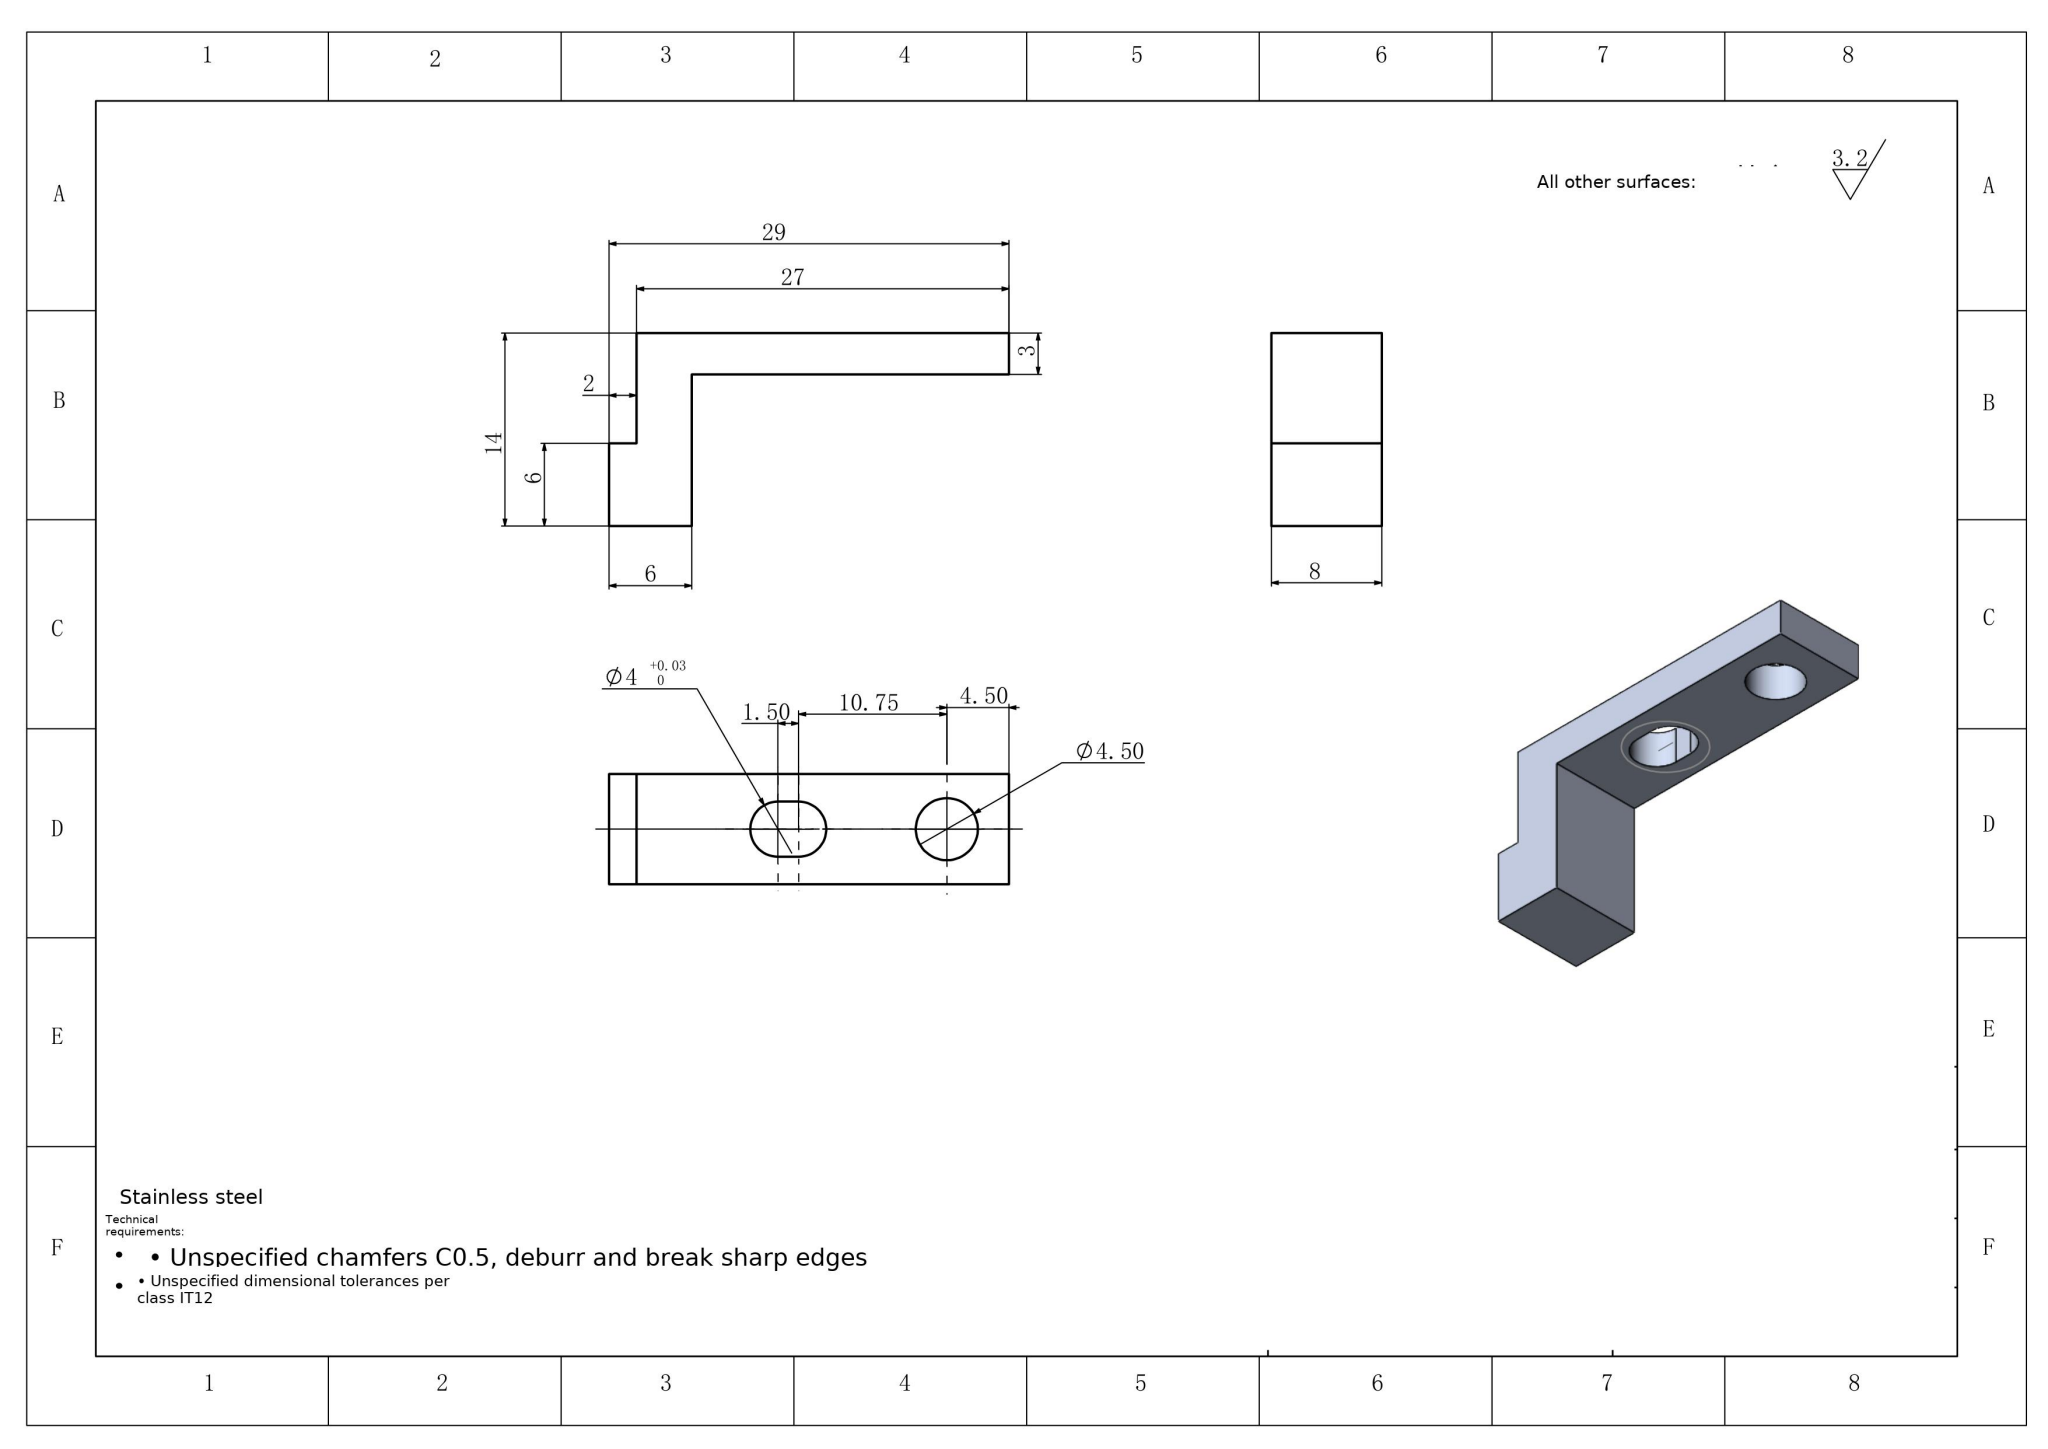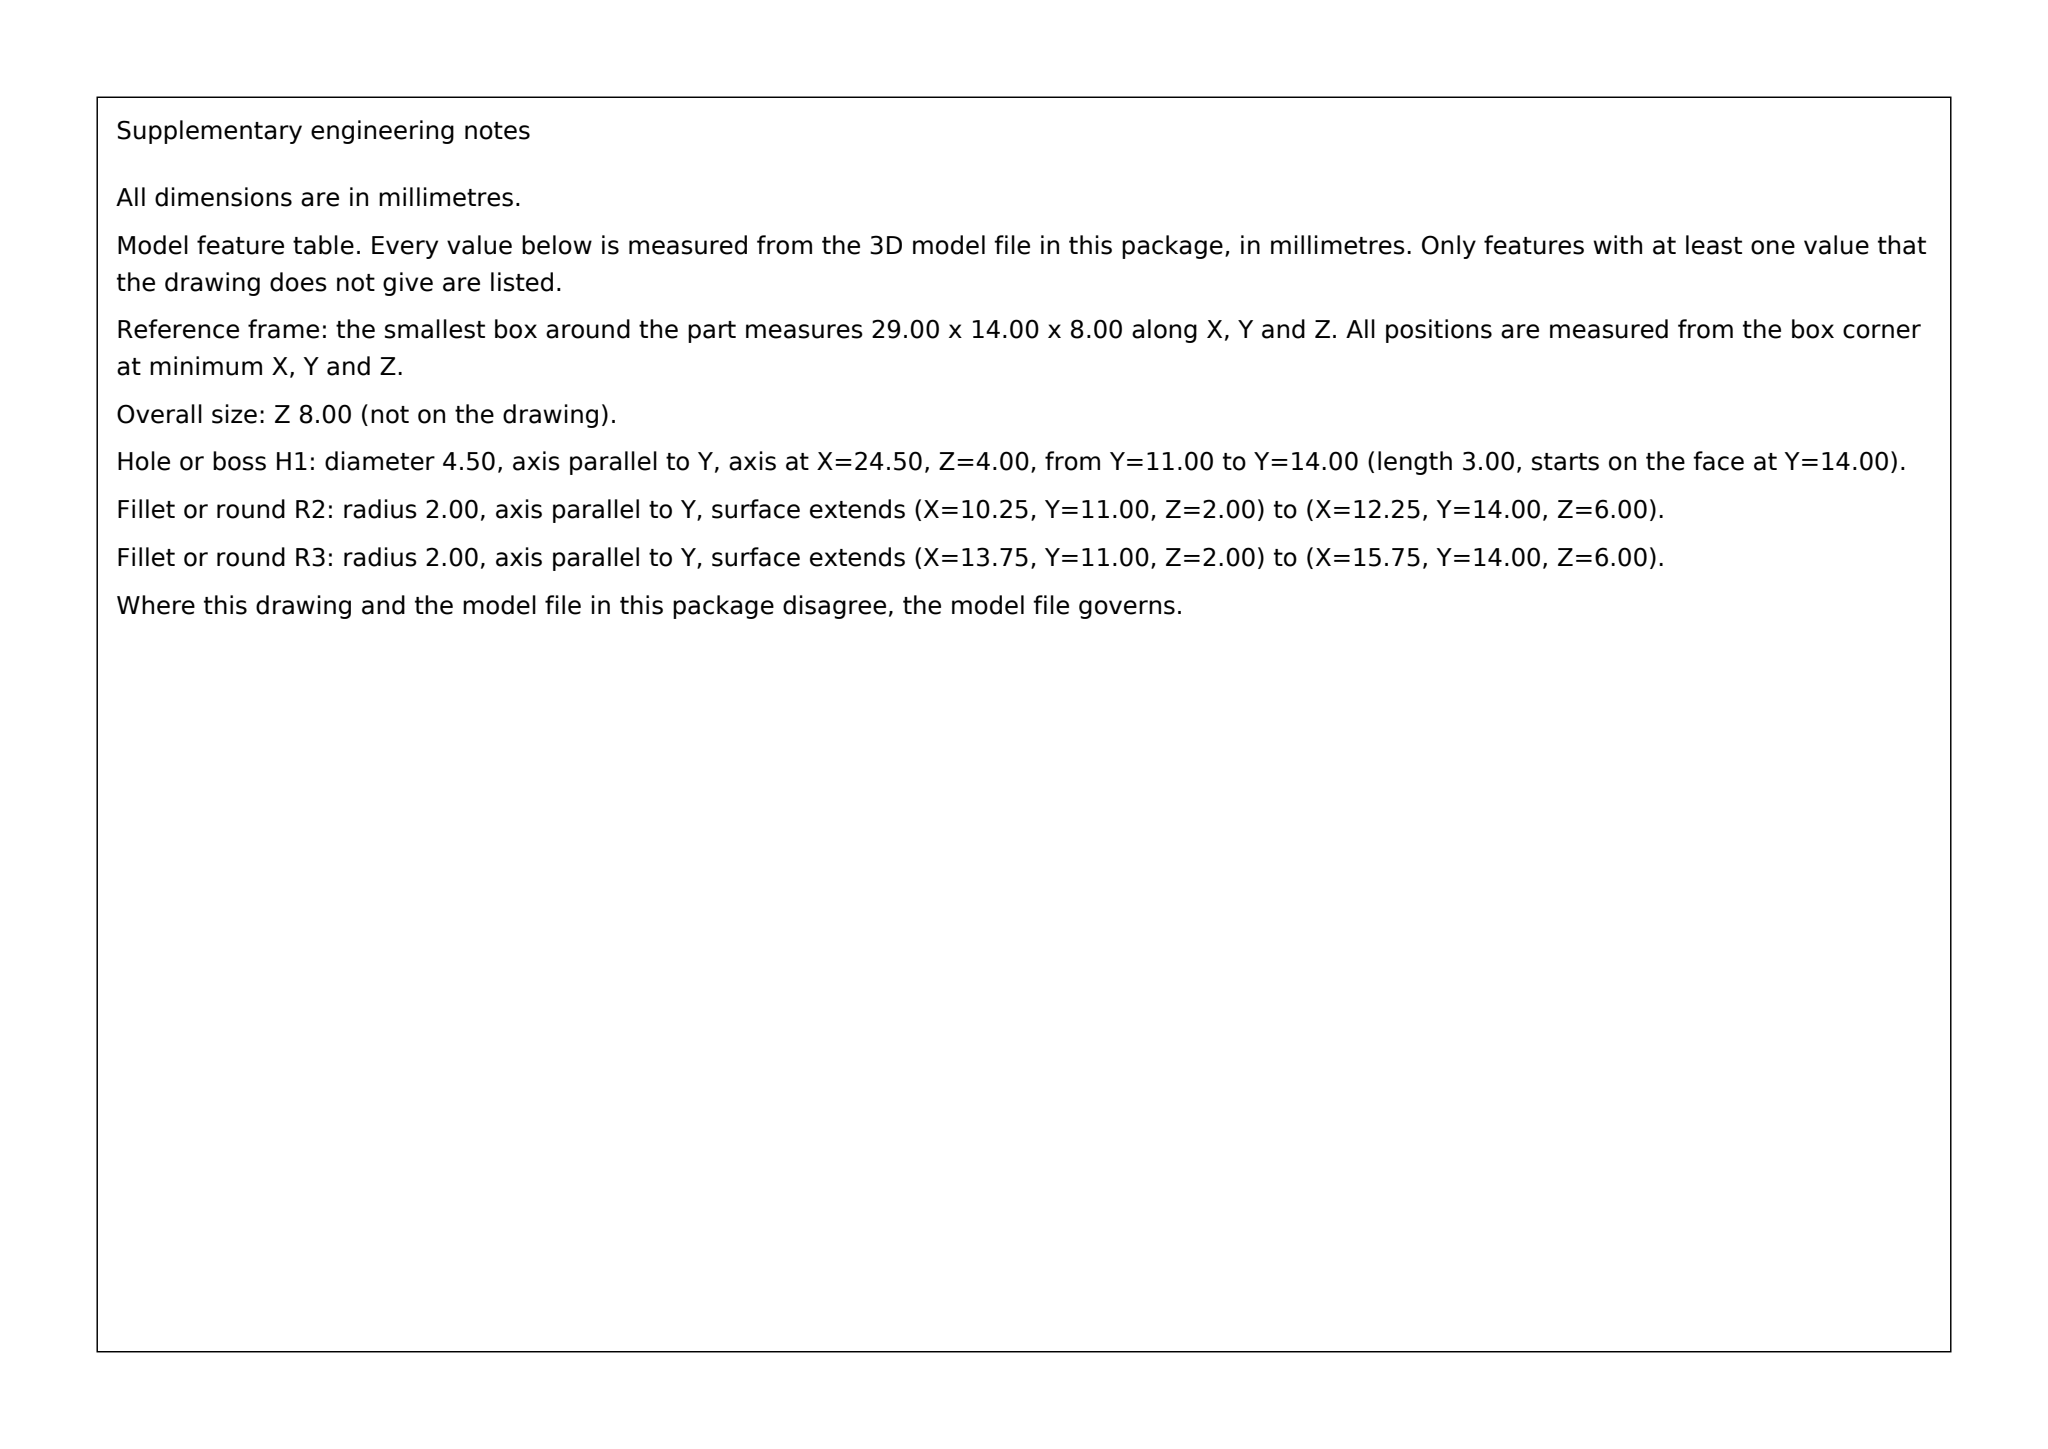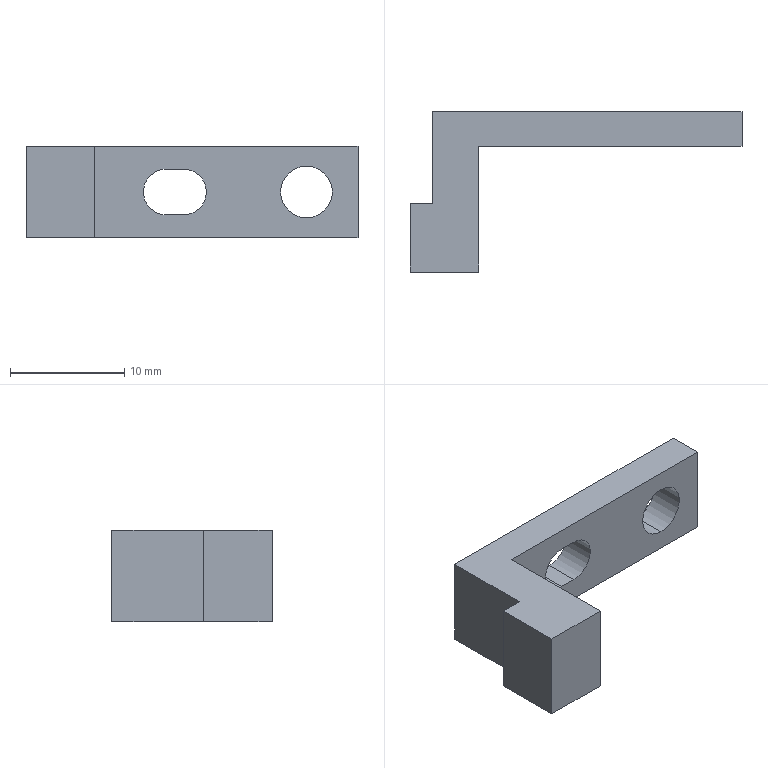Part | SolidWorks | mm | material Stainless steel | 1 solid | 16 faces | box 29 x 14 x 8 mm | volume 993 mm3 | plane 12 | cylinder 4 | commonest cylinder face diameters 4.5 x2 4 x2
build123d program:
from build123d import *

# Parameters (mm, degrees)
BOSS_EXTRUDE1_DEPTH = 4
SKETCH2_R           = 2.25
CUT_EXTRUDE1_DEPTH  = 30.428


with BuildPart() as part:
    # Sketch1 → Boss-Extrude1 (new, symmetric)
    with BuildSketch(Plane.XY):
        Polygon((0, 0), (0, -8), (-2, -8), (-2, -14), (4, -14), (4, -3), (27, -3), (27, 0), align=None)
    extrude(amount=BOSS_EXTRUDE1_DEPTH, both=True)

    # Sketch2 → Cut-Extrude1 (cut, through all)
    with BuildSketch(Plane.XZ.offset(3)):
        with Locations(Location((22.5, 0, 0), (0, 0, 270))):
            Circle(SKETCH2_R)
        with BuildLine():
            Line((10.25, 2), (11.75, 2))
            ThreePointArc((11.75, 2), (13.75, 0), (11.75, -2))
            Line((11.75, -2), (10.25, -2))
            ThreePointArc((10.25, -2), (8.25, 0), (10.25, 2))
        make_face()
    extrude(amount=-CUT_EXTRUDE1_DEPTH, mode=Mode.SUBTRACT)


solid = part.part
STEP:
#1=CARTESIAN_POINT('',(22.5,0.,2.25));
#2=VERTEX_POINT('',#1);
#3=CARTESIAN_POINT('',(22.5,0.,-2.25));
#4=VERTEX_POINT('',#3);
#5=CARTESIAN_POINT('',(22.5,0.,-0.));
#6=DIRECTION('',(0.,-1.,0.));
#7=DIRECTION('',(0.,0.,-1.));
#8=AXIS2_PLACEMENT_3D('',#5,#6,#7);
#9=CIRCLE('',#8,2.25);
#10=EDGE_CURVE('',#2,#4,#9,.T.);
#11=ORIENTED_EDGE('',*,*,#10,.F.);
#12=CARTESIAN_POINT('',(22.5,-3.,2.25));
#13=VERTEX_POINT('',#12);
#14=CARTESIAN_POINT('',(22.5,0.,2.25));
#15=DIRECTION('',(0.,-1.,0.));
#16=VECTOR('',#15,1000.);
#17=LINE('',#14,#16);
#18=EDGE_CURVE('',#2,#13,#17,.T.);
#19=ORIENTED_EDGE('',*,*,#18,.T.);
#20=CARTESIAN_POINT('',(22.5,-3.,-2.25));
#21=VERTEX_POINT('',#20);
#22=CARTESIAN_POINT('',(22.5,-3.,-0.));
#23=DIRECTION('',(0.,-1.,0.));
#24=DIRECTION('',(0.,0.,-1.));
#25=AXIS2_PLACEMENT_3D('',#22,#23,#24);
#26=CIRCLE('',#25,2.25);
#27=EDGE_CURVE('',#13,#21,#26,.T.);
#28=ORIENTED_EDGE('',*,*,#27,.T.);
#29=CARTESIAN_POINT('',(22.5,0.,-2.25));
#30=DIRECTION('',(0.,-1.,0.));
#31=VECTOR('',#30,1000.);
#32=LINE('',#29,#31);
#33=EDGE_CURVE('',#4,#21,#32,.T.);
#34=ORIENTED_EDGE('',*,*,#33,.F.);
#35=EDGE_LOOP('',(#11,#19,#28,#34));
#36=FACE_OUTER_BOUND('',#35,.T.);
#37=CARTESIAN_POINT('',(22.5,0.,-0.));
#38=DIRECTION('',(0.,-1.,0.));
#39=DIRECTION('',(0.,0.,-1.));
#40=AXIS2_PLACEMENT_3D('',#37,#38,#39);
#41=CYLINDRICAL_SURFACE('',#40,2.25);
#42=ADVANCED_FACE('',(#36),#41,.F.);
#43=CARTESIAN_POINT('',(11.75,0.,2.));
#44=VERTEX_POINT('',#43);
#45=CARTESIAN_POINT('',(10.25,0.,2.));
#46=VERTEX_POINT('',#45);
#47=CARTESIAN_POINT('',(10.25,0.,2.));
#48=DIRECTION('',(-1.,0.,-0.));
#49=VECTOR('',#48,1000.);
#50=LINE('',#47,#49);
#51=EDGE_CURVE('',#44,#46,#50,.T.);
#52=ORIENTED_EDGE('',*,*,#51,.T.);
#53=CARTESIAN_POINT('',(10.25,0.,-2.));
#54=VERTEX_POINT('',#53);
#55=CARTESIAN_POINT('',(10.25,0.,-0.));
#56=DIRECTION('',(0.,-1.,0.));
#57=DIRECTION('',(0.,0.,-1.));
#58=AXIS2_PLACEMENT_3D('',#55,#56,#57);
#59=CIRCLE('',#58,2.);
#60=EDGE_CURVE('',#46,#54,#59,.T.);
#61=ORIENTED_EDGE('',*,*,#60,.T.);
#62=CARTESIAN_POINT('',(11.75,0.,-2.));
#63=VERTEX_POINT('',#62);
#64=CARTESIAN_POINT('',(10.25,0.,-2.));
#65=DIRECTION('',(1.,0.,0.));
#66=VECTOR('',#65,1000.);
#67=LINE('',#64,#66);
#68=EDGE_CURVE('',#54,#63,#67,.T.);
#69=ORIENTED_EDGE('',*,*,#68,.T.);
#70=CARTESIAN_POINT('',(11.75,0.,-0.));
#71=DIRECTION('',(0.,-1.,0.));
#72=DIRECTION('',(0.,0.,-1.));
#73=AXIS2_PLACEMENT_3D('',#70,#71,#72);
#74=CIRCLE('',#73,2.);
#75=EDGE_CURVE('',#63,#44,#74,.T.);
#76=ORIENTED_EDGE('',*,*,#75,.T.);
#77=EDGE_LOOP('',(#52,#61,#69,#76));
#78=FACE_BOUND('',#77,.T.);
#79=CARTESIAN_POINT('',(22.5,0.,-0.));
#80=DIRECTION('',(0.,-1.,0.));
#81=DIRECTION('',(0.,0.,-1.));
#82=AXIS2_PLACEMENT_3D('',#79,#80,#81);
#83=CIRCLE('',#82,2.25);
#84=EDGE_CURVE('',#4,#2,#83,.T.);
#85=ORIENTED_EDGE('',*,*,#84,.T.);
#86=ORIENTED_EDGE('',*,*,#10,.T.);
#87=EDGE_LOOP('',(#85,#86));
#88=FACE_BOUND('',#87,.T.);
#89=CARTESIAN_POINT('',(27.,0.,-4.));
#90=VERTEX_POINT('',#89);
#91=CARTESIAN_POINT('',(0.,0.,-4.));
#92=VERTEX_POINT('',#91);
#93=CARTESIAN_POINT('',(27.,0.,-4.));
#94=DIRECTION('',(-1.,-0.,0.));
#95=VECTOR('',#94,1000.);
#96=LINE('',#93,#95);
#97=EDGE_CURVE('',#90,#92,#96,.T.);
#98=ORIENTED_EDGE('',*,*,#97,.T.);
#99=CARTESIAN_POINT('',(0.,0.,4.));
#100=VERTEX_POINT('',#99);
#101=CARTESIAN_POINT('',(0.,0.,4.));
#102=DIRECTION('',(0.,0.,-1.));
#103=VECTOR('',#102,1000.);
#104=LINE('',#101,#103);
#105=EDGE_CURVE('',#100,#92,#104,.T.);
#106=ORIENTED_EDGE('',*,*,#105,.F.);
#107=CARTESIAN_POINT('',(27.,0.,4.));
#108=VERTEX_POINT('',#107);
#109=CARTESIAN_POINT('',(27.,0.,4.));
#110=DIRECTION('',(-1.,-0.,0.));
#111=VECTOR('',#110,1000.);
#112=LINE('',#109,#111);
#113=EDGE_CURVE('',#108,#100,#112,.T.);
#114=ORIENTED_EDGE('',*,*,#113,.F.);
#115=CARTESIAN_POINT('',(27.,0.,4.));
#116=DIRECTION('',(0.,0.,-1.));
#117=VECTOR('',#116,1000.);
#118=LINE('',#115,#117);
#119=EDGE_CURVE('',#108,#90,#118,.T.);
#120=ORIENTED_EDGE('',*,*,#119,.T.);
#121=EDGE_LOOP('',(#98,#106,#114,#120));
#122=FACE_OUTER_BOUND('',#121,.T.);
#123=CARTESIAN_POINT('',(27.,0.,4.));
#124=DIRECTION('',(0.,-1.,0.));
#125=DIRECTION('',(1.,0.,0.));
#126=AXIS2_PLACEMENT_3D('',#123,#124,#125);
#127=PLANE('',#126);
#128=ADVANCED_FACE('',(#78,#88,#122),#127,.F.);
#129=CARTESIAN_POINT('',(0.,-8.,-4.));
#130=VERTEX_POINT('',#129);
#131=CARTESIAN_POINT('',(0.,0.,-4.));
#132=DIRECTION('',(0.,-1.,0.));
#133=VECTOR('',#132,1000.);
#134=LINE('',#131,#133);
#135=EDGE_CURVE('',#92,#130,#134,.T.);
#136=ORIENTED_EDGE('',*,*,#135,.T.);
#137=CARTESIAN_POINT('',(0.,-8.,4.));
#138=VERTEX_POINT('',#137);
#139=CARTESIAN_POINT('',(0.,-8.,4.));
#140=DIRECTION('',(0.,0.,-1.));
#141=VECTOR('',#140,1000.);
#142=LINE('',#139,#141);
#143=EDGE_CURVE('',#138,#130,#142,.T.);
#144=ORIENTED_EDGE('',*,*,#143,.F.);
#145=CARTESIAN_POINT('',(0.,0.,4.));
#146=DIRECTION('',(0.,-1.,0.));
#147=VECTOR('',#146,1000.);
#148=LINE('',#145,#147);
#149=EDGE_CURVE('',#100,#138,#148,.T.);
#150=ORIENTED_EDGE('',*,*,#149,.F.);
#151=ORIENTED_EDGE('',*,*,#105,.T.);
#152=EDGE_LOOP('',(#136,#144,#150,#151));
#153=FACE_OUTER_BOUND('',#152,.T.);
#154=CARTESIAN_POINT('',(0.,0.,4.));
#155=DIRECTION('',(1.,0.,0.));
#156=DIRECTION('',(-0.,1.,0.));
#157=AXIS2_PLACEMENT_3D('',#154,#155,#156);
#158=PLANE('',#157);
#159=ADVANCED_FACE('',(#153),#158,.F.);
#160=CARTESIAN_POINT('',(-2.,-8.,-4.));
#161=VERTEX_POINT('',#160);
#162=CARTESIAN_POINT('',(0.,-8.,-4.));
#163=DIRECTION('',(-1.,0.,0.));
#164=VECTOR('',#163,1000.);
#165=LINE('',#162,#164);
#166=EDGE_CURVE('',#130,#161,#165,.T.);
#167=ORIENTED_EDGE('',*,*,#166,.T.);
#168=CARTESIAN_POINT('',(-2.,-8.,4.));
#169=VERTEX_POINT('',#168);
#170=CARTESIAN_POINT('',(-2.,-8.,4.));
#171=DIRECTION('',(0.,0.,-1.));
#172=VECTOR('',#171,1000.);
#173=LINE('',#170,#172);
#174=EDGE_CURVE('',#169,#161,#173,.T.);
#175=ORIENTED_EDGE('',*,*,#174,.F.);
#176=CARTESIAN_POINT('',(0.,-8.,4.));
#177=DIRECTION('',(-1.,0.,0.));
#178=VECTOR('',#177,1000.);
#179=LINE('',#176,#178);
#180=EDGE_CURVE('',#138,#169,#179,.T.);
#181=ORIENTED_EDGE('',*,*,#180,.F.);
#182=ORIENTED_EDGE('',*,*,#143,.T.);
#183=EDGE_LOOP('',(#167,#175,#181,#182));
#184=FACE_OUTER_BOUND('',#183,.T.);
#185=CARTESIAN_POINT('',(0.,-8.,4.));
#186=DIRECTION('',(0.,-1.,0.));
#187=DIRECTION('',(0.,0.,-1.));
#188=AXIS2_PLACEMENT_3D('',#185,#186,#187);
#189=PLANE('',#188);
#190=ADVANCED_FACE('',(#184),#189,.F.);
#191=CARTESIAN_POINT('',(-2.,-14.,-4.));
#192=VERTEX_POINT('',#191);
#193=CARTESIAN_POINT('',(-2.,-8.,-4.));
#194=DIRECTION('',(0.,-1.,0.));
#195=VECTOR('',#194,1000.);
#196=LINE('',#193,#195);
#197=EDGE_CURVE('',#161,#192,#196,.T.);
#198=ORIENTED_EDGE('',*,*,#197,.T.);
#199=CARTESIAN_POINT('',(-2.,-14.,4.));
#200=VERTEX_POINT('',#199);
#201=CARTESIAN_POINT('',(-2.,-14.,4.));
#202=DIRECTION('',(0.,0.,-1.));
#203=VECTOR('',#202,1000.);
#204=LINE('',#201,#203);
#205=EDGE_CURVE('',#200,#192,#204,.T.);
#206=ORIENTED_EDGE('',*,*,#205,.F.);
#207=CARTESIAN_POINT('',(-2.,-8.,4.));
#208=DIRECTION('',(0.,-1.,0.));
#209=VECTOR('',#208,1000.);
#210=LINE('',#207,#209);
#211=EDGE_CURVE('',#169,#200,#210,.T.);
#212=ORIENTED_EDGE('',*,*,#211,.F.);
#213=ORIENTED_EDGE('',*,*,#174,.T.);
#214=EDGE_LOOP('',(#198,#206,#212,#213));
#215=FACE_OUTER_BOUND('',#214,.T.);
#216=CARTESIAN_POINT('',(-2.,-8.,4.));
#217=DIRECTION('',(1.,0.,0.));
#218=DIRECTION('',(-0.,1.,0.));
#219=AXIS2_PLACEMENT_3D('',#216,#217,#218);
#220=PLANE('',#219);
#221=ADVANCED_FACE('',(#215),#220,.F.);
#222=CARTESIAN_POINT('',(4.,-14.,-4.));
#223=VERTEX_POINT('',#222);
#224=CARTESIAN_POINT('',(-2.,-14.,-4.));
#225=DIRECTION('',(1.,0.,0.));
#226=VECTOR('',#225,1000.);
#227=LINE('',#224,#226);
#228=EDGE_CURVE('',#192,#223,#227,.T.);
#229=ORIENTED_EDGE('',*,*,#228,.T.);
#230=CARTESIAN_POINT('',(4.,-14.,4.));
#231=VERTEX_POINT('',#230);
#232=CARTESIAN_POINT('',(4.,-14.,4.));
#233=DIRECTION('',(0.,0.,-1.));
#234=VECTOR('',#233,1000.);
#235=LINE('',#232,#234);
#236=EDGE_CURVE('',#231,#223,#235,.T.);
#237=ORIENTED_EDGE('',*,*,#236,.F.);
#238=CARTESIAN_POINT('',(-2.,-14.,4.));
#239=DIRECTION('',(1.,0.,0.));
#240=VECTOR('',#239,1000.);
#241=LINE('',#238,#240);
#242=EDGE_CURVE('',#200,#231,#241,.T.);
#243=ORIENTED_EDGE('',*,*,#242,.F.);
#244=ORIENTED_EDGE('',*,*,#205,.T.);
#245=EDGE_LOOP('',(#229,#237,#243,#244));
#246=FACE_OUTER_BOUND('',#245,.T.);
#247=CARTESIAN_POINT('',(-2.,-14.,4.));
#248=DIRECTION('',(0.,1.,0.));
#249=DIRECTION('',(0.,0.,1.));
#250=AXIS2_PLACEMENT_3D('',#247,#248,#249);
#251=PLANE('',#250);
#252=ADVANCED_FACE('',(#246),#251,.F.);
#253=CARTESIAN_POINT('',(4.,-3.,-4.));
#254=VERTEX_POINT('',#253);
#255=CARTESIAN_POINT('',(4.,-14.,-4.));
#256=DIRECTION('',(0.,1.,0.));
#257=VECTOR('',#256,1000.);
#258=LINE('',#255,#257);
#259=EDGE_CURVE('',#223,#254,#258,.T.);
#260=ORIENTED_EDGE('',*,*,#259,.T.);
#261=CARTESIAN_POINT('',(4.,-3.,4.));
#262=VERTEX_POINT('',#261);
#263=CARTESIAN_POINT('',(4.,-3.,4.));
#264=DIRECTION('',(0.,0.,-1.));
#265=VECTOR('',#264,1000.);
#266=LINE('',#263,#265);
#267=EDGE_CURVE('',#262,#254,#266,.T.);
#268=ORIENTED_EDGE('',*,*,#267,.F.);
#269=CARTESIAN_POINT('',(4.,-14.,4.));
#270=DIRECTION('',(0.,1.,0.));
#271=VECTOR('',#270,1000.);
#272=LINE('',#269,#271);
#273=EDGE_CURVE('',#231,#262,#272,.T.);
#274=ORIENTED_EDGE('',*,*,#273,.F.);
#275=ORIENTED_EDGE('',*,*,#236,.T.);
#276=EDGE_LOOP('',(#260,#268,#274,#275));
#277=FACE_OUTER_BOUND('',#276,.T.);
#278=CARTESIAN_POINT('',(4.,-14.,4.));
#279=DIRECTION('',(-1.,0.,0.));
#280=DIRECTION('',(0.,0.,1.));
#281=AXIS2_PLACEMENT_3D('',#278,#279,#280);
#282=PLANE('',#281);
#283=ADVANCED_FACE('',(#277),#282,.F.);
#284=CARTESIAN_POINT('',(10.25,-3.,-2.));
#285=VERTEX_POINT('',#284);
#286=CARTESIAN_POINT('',(11.75,-3.,-2.));
#287=VERTEX_POINT('',#286);
#288=CARTESIAN_POINT('',(10.25,-3.,-2.));
#289=DIRECTION('',(1.,0.,0.));
#290=VECTOR('',#289,1000.);
#291=LINE('',#288,#290);
#292=EDGE_CURVE('',#285,#287,#291,.T.);
#293=ORIENTED_EDGE('',*,*,#292,.F.);
#294=CARTESIAN_POINT('',(10.25,-3.,2.));
#295=VERTEX_POINT('',#294);
#296=CARTESIAN_POINT('',(10.25,-3.,-0.));
#297=DIRECTION('',(0.,-1.,0.));
#298=DIRECTION('',(0.,0.,-1.));
#299=AXIS2_PLACEMENT_3D('',#296,#297,#298);
#300=CIRCLE('',#299,2.);
#301=EDGE_CURVE('',#295,#285,#300,.T.);
#302=ORIENTED_EDGE('',*,*,#301,.F.);
#303=CARTESIAN_POINT('',(11.75,-3.,2.));
#304=VERTEX_POINT('',#303);
#305=CARTESIAN_POINT('',(10.25,-3.,2.));
#306=DIRECTION('',(-1.,0.,-0.));
#307=VECTOR('',#306,1000.);
#308=LINE('',#305,#307);
#309=EDGE_CURVE('',#304,#295,#308,.T.);
#310=ORIENTED_EDGE('',*,*,#309,.F.);
#311=CARTESIAN_POINT('',(11.75,-3.,-0.));
#312=DIRECTION('',(0.,-1.,0.));
#313=DIRECTION('',(0.,0.,-1.));
#314=AXIS2_PLACEMENT_3D('',#311,#312,#313);
#315=CIRCLE('',#314,2.);
#316=EDGE_CURVE('',#287,#304,#315,.T.);
#317=ORIENTED_EDGE('',*,*,#316,.F.);
#318=EDGE_LOOP('',(#293,#302,#310,#317));
#319=FACE_BOUND('',#318,.T.);
#320=CARTESIAN_POINT('',(22.5,-3.,-0.));
#321=DIRECTION('',(0.,-1.,0.));
#322=DIRECTION('',(0.,0.,-1.));
#323=AXIS2_PLACEMENT_3D('',#320,#321,#322);
#324=CIRCLE('',#323,2.25);
#325=EDGE_CURVE('',#21,#13,#324,.T.);
#326=ORIENTED_EDGE('',*,*,#325,.F.);
#327=ORIENTED_EDGE('',*,*,#27,.F.);
#328=EDGE_LOOP('',(#326,#327));
#329=FACE_BOUND('',#328,.T.);
#330=CARTESIAN_POINT('',(27.,-3.,-4.));
#331=VERTEX_POINT('',#330);
#332=CARTESIAN_POINT('',(4.,-3.,-4.));
#333=DIRECTION('',(1.,0.,0.));
#334=VECTOR('',#333,1000.);
#335=LINE('',#332,#334);
#336=EDGE_CURVE('',#254,#331,#335,.T.);
#337=ORIENTED_EDGE('',*,*,#336,.T.);
#338=CARTESIAN_POINT('',(27.,-3.,4.));
#339=VERTEX_POINT('',#338);
#340=CARTESIAN_POINT('',(27.,-3.,4.));
#341=DIRECTION('',(0.,0.,-1.));
#342=VECTOR('',#341,1000.);
#343=LINE('',#340,#342);
#344=EDGE_CURVE('',#339,#331,#343,.T.);
#345=ORIENTED_EDGE('',*,*,#344,.F.);
#346=CARTESIAN_POINT('',(4.,-3.,4.));
#347=DIRECTION('',(1.,0.,0.));
#348=VECTOR('',#347,1000.);
#349=LINE('',#346,#348);
#350=EDGE_CURVE('',#262,#339,#349,.T.);
#351=ORIENTED_EDGE('',*,*,#350,.F.);
#352=ORIENTED_EDGE('',*,*,#267,.T.);
#353=EDGE_LOOP('',(#337,#345,#351,#352));
#354=FACE_OUTER_BOUND('',#353,.T.);
#355=CARTESIAN_POINT('',(4.,-3.,4.));
#356=DIRECTION('',(-0.,1.,0.));
#357=DIRECTION('',(-1.,-0.,0.));
#358=AXIS2_PLACEMENT_3D('',#355,#356,#357);
#359=PLANE('',#358);
#360=ADVANCED_FACE('',(#319,#329,#354),#359,.F.);
#361=CARTESIAN_POINT('',(27.,-3.,-4.));
#362=DIRECTION('',(0.,1.,0.));
#363=VECTOR('',#362,1000.);
#364=LINE('',#361,#363);
#365=EDGE_CURVE('',#331,#90,#364,.T.);
#366=ORIENTED_EDGE('',*,*,#365,.T.);
#367=ORIENTED_EDGE('',*,*,#119,.F.);
#368=CARTESIAN_POINT('',(27.,-3.,4.));
#369=DIRECTION('',(0.,1.,0.));
#370=VECTOR('',#369,1000.);
#371=LINE('',#368,#370);
#372=EDGE_CURVE('',#339,#108,#371,.T.);
#373=ORIENTED_EDGE('',*,*,#372,.F.);
#374=ORIENTED_EDGE('',*,*,#344,.T.);
#375=EDGE_LOOP('',(#366,#367,#373,#374));
#376=FACE_OUTER_BOUND('',#375,.T.);
#377=CARTESIAN_POINT('',(27.,-3.,4.));
#378=DIRECTION('',(-1.,0.,0.));
#379=DIRECTION('',(0.,0.,1.));
#380=AXIS2_PLACEMENT_3D('',#377,#378,#379);
#381=PLANE('',#380);
#382=ADVANCED_FACE('',(#376),#381,.F.);
#383=ORIENTED_EDGE('',*,*,#113,.T.);
#384=ORIENTED_EDGE('',*,*,#149,.T.);
#385=ORIENTED_EDGE('',*,*,#180,.T.);
#386=ORIENTED_EDGE('',*,*,#211,.T.);
#387=ORIENTED_EDGE('',*,*,#242,.T.);
#388=ORIENTED_EDGE('',*,*,#273,.T.);
#389=ORIENTED_EDGE('',*,*,#350,.T.);
#390=ORIENTED_EDGE('',*,*,#372,.T.);
#391=EDGE_LOOP('',(#383,#384,#385,#386,#387,#388,#389,#390));
#392=FACE_OUTER_BOUND('',#391,.T.);
#393=CARTESIAN_POINT('',(0.,0.,4.));
#394=DIRECTION('',(0.,0.,1.));
#395=DIRECTION('',(1.,0.,0.));
#396=AXIS2_PLACEMENT_3D('',#393,#394,#395);
#397=PLANE('',#396);
#398=ADVANCED_FACE('',(#392),#397,.T.);
#399=ORIENTED_EDGE('',*,*,#97,.F.);
#400=ORIENTED_EDGE('',*,*,#365,.F.);
#401=ORIENTED_EDGE('',*,*,#336,.F.);
#402=ORIENTED_EDGE('',*,*,#259,.F.);
#403=ORIENTED_EDGE('',*,*,#228,.F.);
#404=ORIENTED_EDGE('',*,*,#197,.F.);
#405=ORIENTED_EDGE('',*,*,#166,.F.);
#406=ORIENTED_EDGE('',*,*,#135,.F.);
#407=EDGE_LOOP('',(#399,#400,#401,#402,#403,#404,#405,#406));
#408=FACE_OUTER_BOUND('',#407,.T.);
#409=CARTESIAN_POINT('',(0.,0.,-4.));
#410=DIRECTION('',(0.,0.,1.));
#411=DIRECTION('',(1.,0.,0.));
#412=AXIS2_PLACEMENT_3D('',#409,#410,#411);
#413=PLANE('',#412);
#414=ADVANCED_FACE('',(#408),#413,.F.);
#415=ORIENTED_EDGE('',*,*,#18,.F.);
#416=ORIENTED_EDGE('',*,*,#84,.F.);
#417=ORIENTED_EDGE('',*,*,#33,.T.);
#418=ORIENTED_EDGE('',*,*,#325,.T.);
#419=EDGE_LOOP('',(#415,#416,#417,#418));
#420=FACE_OUTER_BOUND('',#419,.T.);
#421=CARTESIAN_POINT('',(22.5,0.,-0.));
#422=DIRECTION('',(0.,-1.,0.));
#423=DIRECTION('',(0.,0.,-1.));
#424=AXIS2_PLACEMENT_3D('',#421,#422,#423);
#425=CYLINDRICAL_SURFACE('',#424,2.25);
#426=ADVANCED_FACE('',(#420),#425,.F.);
#427=ORIENTED_EDGE('',*,*,#301,.T.);
#428=CARTESIAN_POINT('',(10.25,0.,-2.));
#429=DIRECTION('',(0.,-1.,0.));
#430=VECTOR('',#429,1000.);
#431=LINE('',#428,#430);
#432=EDGE_CURVE('',#54,#285,#431,.T.);
#433=ORIENTED_EDGE('',*,*,#432,.F.);
#434=ORIENTED_EDGE('',*,*,#60,.F.);
#435=CARTESIAN_POINT('',(10.25,0.,2.));
#436=DIRECTION('',(0.,-1.,0.));
#437=VECTOR('',#436,1000.);
#438=LINE('',#435,#437);
#439=EDGE_CURVE('',#46,#295,#438,.T.);
#440=ORIENTED_EDGE('',*,*,#439,.T.);
#441=EDGE_LOOP('',(#427,#433,#434,#440));
#442=FACE_OUTER_BOUND('',#441,.T.);
#443=CARTESIAN_POINT('',(10.25,0.,-0.));
#444=DIRECTION('',(0.,-1.,0.));
#445=DIRECTION('',(0.,0.,-1.));
#446=AXIS2_PLACEMENT_3D('',#443,#444,#445);
#447=CYLINDRICAL_SURFACE('',#446,2.);
#448=ADVANCED_FACE('',(#442),#447,.F.);
#449=ORIENTED_EDGE('',*,*,#309,.T.);
#450=ORIENTED_EDGE('',*,*,#439,.F.);
#451=ORIENTED_EDGE('',*,*,#51,.F.);
#452=CARTESIAN_POINT('',(11.75,0.,2.));
#453=DIRECTION('',(0.,-1.,0.));
#454=VECTOR('',#453,1000.);
#455=LINE('',#452,#454);
#456=EDGE_CURVE('',#44,#304,#455,.T.);
#457=ORIENTED_EDGE('',*,*,#456,.T.);
#458=EDGE_LOOP('',(#449,#450,#451,#457));
#459=FACE_OUTER_BOUND('',#458,.T.);
#460=CARTESIAN_POINT('',(10.25,0.,2.));
#461=DIRECTION('',(-0.,0.,1.));
#462=DIRECTION('',(1.,0.,0.));
#463=AXIS2_PLACEMENT_3D('',#460,#461,#462);
#464=PLANE('',#463);
#465=ADVANCED_FACE('',(#459),#464,.F.);
#466=ORIENTED_EDGE('',*,*,#316,.T.);
#467=ORIENTED_EDGE('',*,*,#456,.F.);
#468=ORIENTED_EDGE('',*,*,#75,.F.);
#469=CARTESIAN_POINT('',(11.75,0.,-2.));
#470=DIRECTION('',(0.,-1.,0.));
#471=VECTOR('',#470,1000.);
#472=LINE('',#469,#471);
#473=EDGE_CURVE('',#63,#287,#472,.T.);
#474=ORIENTED_EDGE('',*,*,#473,.T.);
#475=EDGE_LOOP('',(#466,#467,#468,#474));
#476=FACE_OUTER_BOUND('',#475,.T.);
#477=CARTESIAN_POINT('',(11.75,0.,-0.));
#478=DIRECTION('',(0.,-1.,0.));
#479=DIRECTION('',(0.,0.,-1.));
#480=AXIS2_PLACEMENT_3D('',#477,#478,#479);
#481=CYLINDRICAL_SURFACE('',#480,2.);
#482=ADVANCED_FACE('',(#476),#481,.F.);
#483=ORIENTED_EDGE('',*,*,#292,.T.);
#484=ORIENTED_EDGE('',*,*,#473,.F.);
#485=ORIENTED_EDGE('',*,*,#68,.F.);
#486=ORIENTED_EDGE('',*,*,#432,.T.);
#487=EDGE_LOOP('',(#483,#484,#485,#486));
#488=FACE_OUTER_BOUND('',#487,.T.);
#489=CARTESIAN_POINT('',(10.25,0.,-2.));
#490=DIRECTION('',(0.,0.,-1.));
#491=DIRECTION('',(-1.,0.,-0.));
#492=AXIS2_PLACEMENT_3D('',#489,#490,#491);
#493=PLANE('',#492);
#494=ADVANCED_FACE('',(#488),#493,.F.);
#495=CLOSED_SHELL('',(#42,#128,#159,#190,#221,#252,#283,#360,#382,#398,#414,#426,#448,#465,#482,#494));
#496=MANIFOLD_SOLID_BREP('',#495);
#497=CARTESIAN_POINT('',(0.,0.,0.));
#498=DIRECTION('',(0.,0.,1.));
#499=DIRECTION('',(1.,0.,0.));
#500=AXIS2_PLACEMENT_3D('',#497,#498,#499);
#501=(LENGTH_UNIT()NAMED_UNIT(*)SI_UNIT(.MILLI.,.METRE.));
#502=UNCERTAINTY_MEASURE_WITH_UNIT(LENGTH_MEASURE(0.00001),#501,'','');
#503=(NAMED_UNIT(*)PLANE_ANGLE_UNIT()SI_UNIT($,.RADIAN.));
#504=(NAMED_UNIT(*)SI_UNIT($,.STERADIAN.)SOLID_ANGLE_UNIT());
#505=(GEOMETRIC_REPRESENTATION_CONTEXT(3)GLOBAL_UNCERTAINTY_ASSIGNED_CONTEXT((#502))GLOBAL_UNIT_ASSIGNED_CONTEXT((#501,#503,#504))REPRESENTATION_CONTEXT('',''));
#506=ADVANCED_BREP_SHAPE_REPRESENTATION('',(#496,#500),#505);